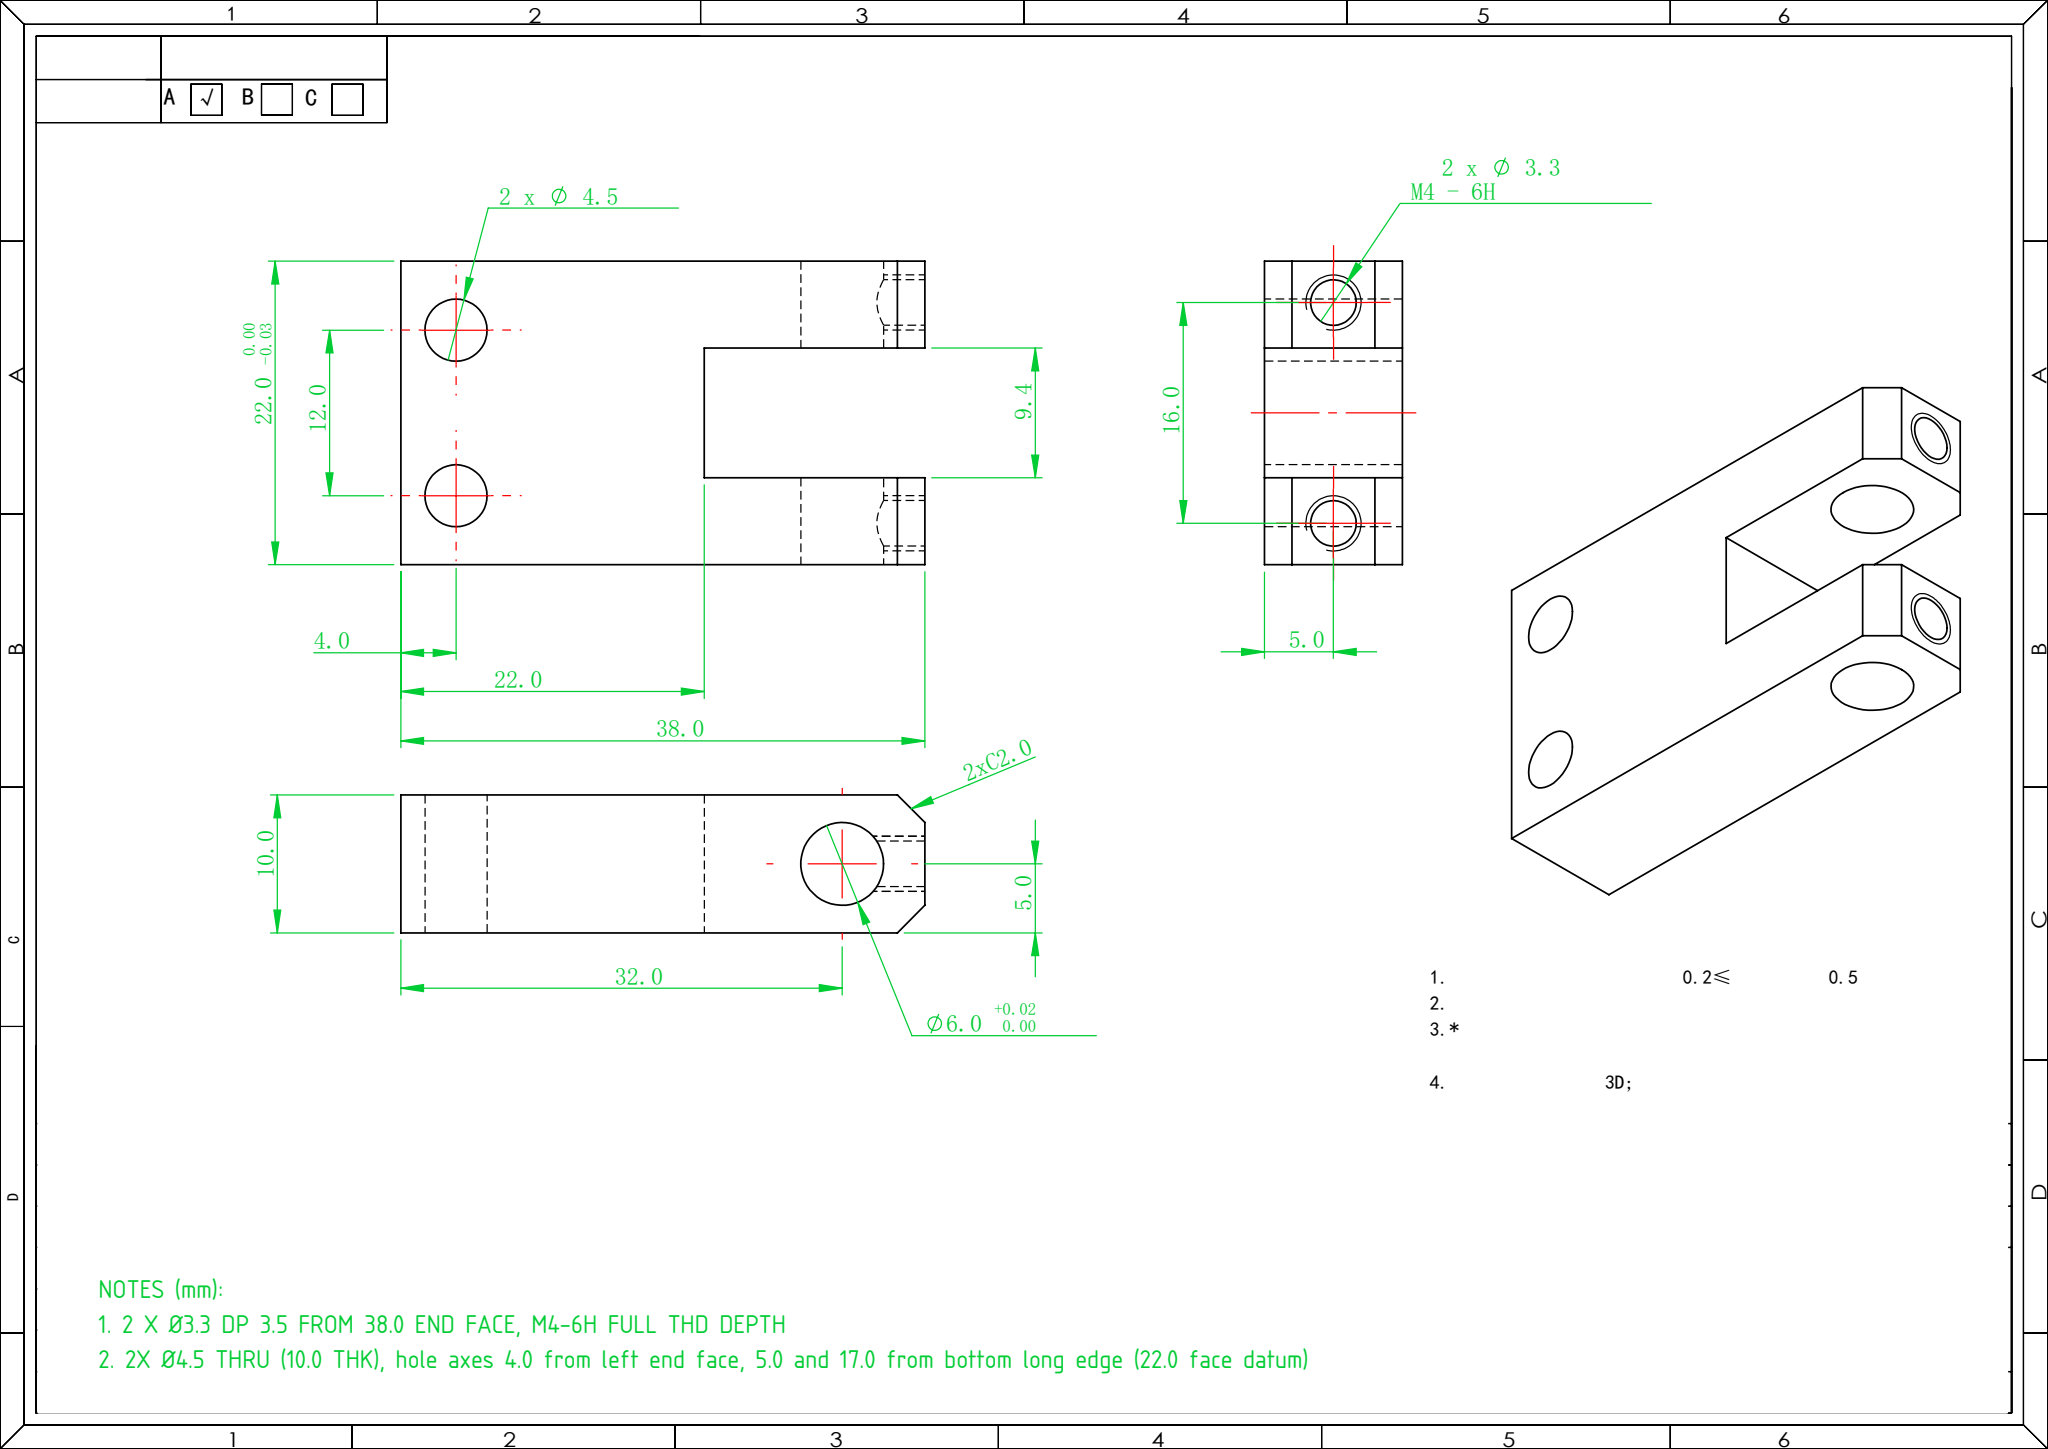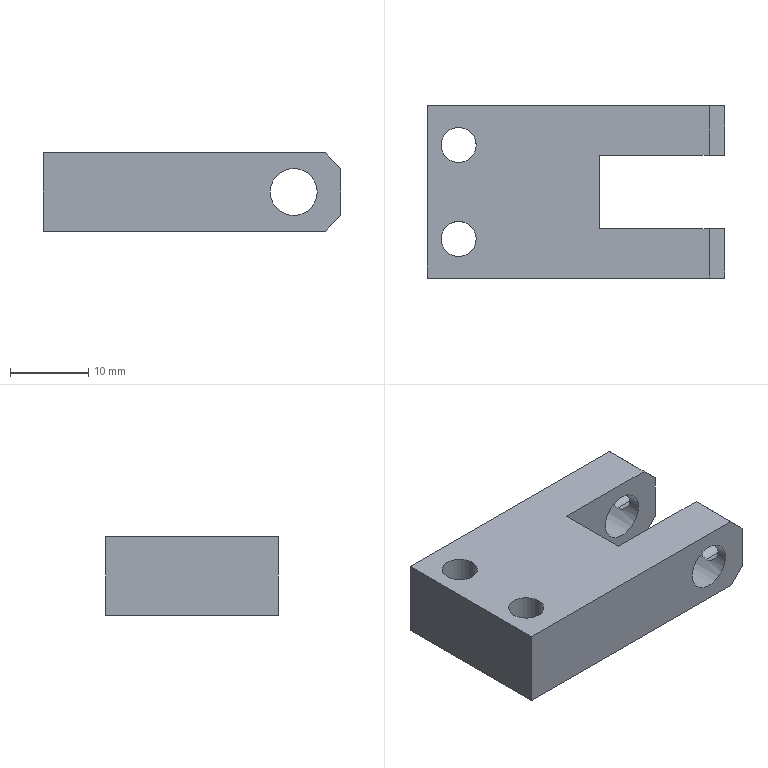Part | SolidWorks | mm | 1 solid | 26 faces | box 38 x 22 x 10 mm | volume 6078 mm3 | plane 14 | cylinder 12 | commonest cylinder face diameters 4.5 x4 3.3 x4 6 x4
Drawing notes:
2 X Ø3.3 DP 3.5 FROM 38.0 END FACE, M4-6H FULL THD DEPTH | from the solid: cylinders [3.3,"x",[null,3.0,5.0],3.49] and [3.3,"x",[null,19.0,5.0],3.49]; blind from x=38.0 face
2X Ø4.5 THRU (10.0 THK), hole axes 4.0 from left end face, 5.0 and 17.0 from bottom long edge (22.0 face datum) | from the solid: cylinders [4.5, axis z, pos (4.0, 5.0) and (4.0, 17.0), length 10.0] with bbox_xyz z = 10.0
STEP:
#1=CARTESIAN_POINT('',(-12.75,-6.,0.));
#2=VERTEX_POINT('',#1);
#3=CARTESIAN_POINT('',(-17.25,-6.,0.));
#4=VERTEX_POINT('',#3);
#5=CARTESIAN_POINT('',(-15.,-6.,0.));
#6=DIRECTION('',(0.,0.,-1.));
#7=DIRECTION('',(-1.,0.,0.));
#8=AXIS2_PLACEMENT_3D('',#5,#6,#7);
#9=CIRCLE('',#8,2.25);
#10=EDGE_CURVE('',#2,#4,#9,.T.);
#11=ORIENTED_EDGE('',*,*,#10,.T.);
#12=CARTESIAN_POINT('',(-17.25,-6.,10.));
#13=VERTEX_POINT('',#12);
#14=CARTESIAN_POINT('',(-17.25,-6.,10.));
#15=DIRECTION('',(0.,0.,1.));
#16=VECTOR('',#15,1000.);
#17=LINE('',#14,#16);
#18=EDGE_CURVE('',#4,#13,#17,.T.);
#19=ORIENTED_EDGE('',*,*,#18,.T.);
#20=CARTESIAN_POINT('',(-12.75,-6.,10.));
#21=VERTEX_POINT('',#20);
#22=CARTESIAN_POINT('',(-15.,-6.,10.));
#23=DIRECTION('',(0.,0.,1.));
#24=DIRECTION('',(1.,0.,0.));
#25=AXIS2_PLACEMENT_3D('',#22,#23,#24);
#26=CIRCLE('',#25,2.25);
#27=EDGE_CURVE('',#13,#21,#26,.T.);
#28=ORIENTED_EDGE('',*,*,#27,.T.);
#29=CARTESIAN_POINT('',(-12.75,-6.,10.));
#30=DIRECTION('',(0.,0.,1.));
#31=VECTOR('',#30,1000.);
#32=LINE('',#29,#31);
#33=EDGE_CURVE('',#2,#21,#32,.T.);
#34=ORIENTED_EDGE('',*,*,#33,.F.);
#35=EDGE_LOOP('',(#11,#19,#28,#34));
#36=FACE_OUTER_BOUND('',#35,.T.);
#37=CARTESIAN_POINT('',(-15.,-6.,10.));
#38=DIRECTION('',(0.,0.,1.));
#39=DIRECTION('',(1.,0.,0.));
#40=AXIS2_PLACEMENT_3D('',#37,#38,#39);
#41=CYLINDRICAL_SURFACE('',#40,2.25);
#42=ADVANCED_FACE('',(#36),#41,.F.);
#43=CARTESIAN_POINT('',(-12.75,6.,0.));
#44=VERTEX_POINT('',#43);
#45=CARTESIAN_POINT('',(-17.25,6.,0.));
#46=VERTEX_POINT('',#45);
#47=CARTESIAN_POINT('',(-15.,6.,0.));
#48=DIRECTION('',(0.,0.,-1.));
#49=DIRECTION('',(-1.,0.,0.));
#50=AXIS2_PLACEMENT_3D('',#47,#48,#49);
#51=CIRCLE('',#50,2.25);
#52=EDGE_CURVE('',#44,#46,#51,.T.);
#53=ORIENTED_EDGE('',*,*,#52,.T.);
#54=CARTESIAN_POINT('',(-17.25,6.,10.));
#55=VERTEX_POINT('',#54);
#56=CARTESIAN_POINT('',(-17.25,6.,10.));
#57=DIRECTION('',(0.,0.,1.));
#58=VECTOR('',#57,1000.);
#59=LINE('',#56,#58);
#60=EDGE_CURVE('',#46,#55,#59,.T.);
#61=ORIENTED_EDGE('',*,*,#60,.T.);
#62=CARTESIAN_POINT('',(-12.75,6.,10.));
#63=VERTEX_POINT('',#62);
#64=CARTESIAN_POINT('',(-15.,6.,10.));
#65=DIRECTION('',(0.,0.,1.));
#66=DIRECTION('',(1.,0.,0.));
#67=AXIS2_PLACEMENT_3D('',#64,#65,#66);
#68=CIRCLE('',#67,2.25);
#69=EDGE_CURVE('',#55,#63,#68,.T.);
#70=ORIENTED_EDGE('',*,*,#69,.T.);
#71=CARTESIAN_POINT('',(-12.75,6.,10.));
#72=DIRECTION('',(0.,0.,1.));
#73=VECTOR('',#72,1000.);
#74=LINE('',#71,#73);
#75=EDGE_CURVE('',#44,#63,#74,.T.);
#76=ORIENTED_EDGE('',*,*,#75,.F.);
#77=EDGE_LOOP('',(#53,#61,#70,#76));
#78=FACE_OUTER_BOUND('',#77,.T.);
#79=CARTESIAN_POINT('',(-15.,6.,10.));
#80=DIRECTION('',(0.,0.,1.));
#81=DIRECTION('',(1.,0.,0.));
#82=AXIS2_PLACEMENT_3D('',#79,#80,#81);
#83=CYLINDRICAL_SURFACE('',#82,2.25);
#84=ADVANCED_FACE('',(#78),#83,.F.);
#85=CARTESIAN_POINT('',(15.505,-8.,6.65));
#86=VERTEX_POINT('',#85);
#87=CARTESIAN_POINT('',(16.,-9.65,5.));
#88=VERTEX_POINT('',#87);
#89=CARTESIAN_POINT('',(15.505,-8.,6.65));
#90=CARTESIAN_POINT('',(15.505,-8.11,6.65));
#91=CARTESIAN_POINT('',(15.513,-8.222,6.639));
#92=CARTESIAN_POINT('',(15.541,-8.436,6.595));
#93=CARTESIAN_POINT('',(15.561,-8.541,6.563));
#94=CARTESIAN_POINT('',(15.635,-8.839,6.437));
#95=CARTESIAN_POINT('',(15.701,-9.018,6.316));
#96=CARTESIAN_POINT('',(15.827,-9.316,6.018));
#97=CARTESIAN_POINT('',(15.888,-9.438,5.837));
#98=CARTESIAN_POINT('',(15.953,-9.563,5.54));
#99=CARTESIAN_POINT('',(15.97,-9.596,5.434));
#100=CARTESIAN_POINT('',(15.994,-9.639,5.219));
#101=CARTESIAN_POINT('',(16.,-9.65,5.11));
#102=CARTESIAN_POINT('',(16.,-9.65,5.));
#103=B_SPLINE_CURVE_WITH_KNOTS('',3,(#89,#90,#91,#92,#93,#94,#95,#96,#97,#98,#99,#100,#101,#102),.UNSPECIFIED.,.F.,.F.,(4,2,2,2,2,2,4),(0.002637,0.002966,0.003296,0.003954,0.004612,0.004941,0.00527),.UNSPECIFIED.);
#104=EDGE_CURVE('',#86,#88,#103,.T.);
#105=ORIENTED_EDGE('',*,*,#104,.F.);
#106=CARTESIAN_POINT('',(19.,-8.,6.65));
#107=VERTEX_POINT('',#106);
#108=CARTESIAN_POINT('',(19.,-8.,6.65));
#109=DIRECTION('',(1.,0.,0.));
#110=VECTOR('',#109,1000.);
#111=LINE('',#108,#110);
#112=EDGE_CURVE('',#86,#107,#111,.T.);
#113=ORIENTED_EDGE('',*,*,#112,.T.);
#114=CARTESIAN_POINT('',(19.,-8.,3.35));
#115=VERTEX_POINT('',#114);
#116=CARTESIAN_POINT('',(19.,-8.,5.));
#117=DIRECTION('',(1.,0.,0.));
#118=DIRECTION('',(0.,0.,-1.));
#119=AXIS2_PLACEMENT_3D('',#116,#117,#118);
#120=CIRCLE('',#119,1.65);
#121=EDGE_CURVE('',#107,#115,#120,.T.);
#122=ORIENTED_EDGE('',*,*,#121,.T.);
#123=CARTESIAN_POINT('',(15.505,-8.,3.35));
#124=VERTEX_POINT('',#123);
#125=CARTESIAN_POINT('',(19.,-8.,3.35));
#126=DIRECTION('',(1.,0.,0.));
#127=VECTOR('',#126,1000.);
#128=LINE('',#125,#127);
#129=EDGE_CURVE('',#124,#115,#128,.T.);
#130=ORIENTED_EDGE('',*,*,#129,.F.);
#131=CARTESIAN_POINT('',(16.,-9.65,5.));
#132=CARTESIAN_POINT('',(16.,-9.65,4.89));
#133=CARTESIAN_POINT('',(15.994,-9.639,4.778));
#134=CARTESIAN_POINT('',(15.97,-9.595,4.564));
#135=CARTESIAN_POINT('',(15.953,-9.563,4.459));
#136=CARTESIAN_POINT('',(15.909,-9.478,4.258));
#137=CARTESIAN_POINT('',(15.883,-9.427,4.164));
#138=CARTESIAN_POINT('',(15.826,-9.307,3.988));
#139=CARTESIAN_POINT('',(15.794,-9.239,3.905));
#140=CARTESIAN_POINT('',(15.7,-9.014,3.682));
#141=CARTESIAN_POINT('',(15.634,-8.834,3.561));
#142=CARTESIAN_POINT('',(15.537,-8.44,3.396));
#143=CARTESIAN_POINT('',(15.505,-8.219,3.35));
#144=CARTESIAN_POINT('',(15.505,-8.,3.35));
#145=B_SPLINE_CURVE_WITH_KNOTS('',3,(#131,#132,#133,#134,#135,#136,#137,#138,#139,#140,#141,#142,#143,#144),.UNSPECIFIED.,.F.,.F.,(4,2,2,2,2,2,4),(0.00527,0.005599,0.005928,0.006257,0.006586,0.007244,0.007902),.UNSPECIFIED.);
#146=EDGE_CURVE('',#88,#124,#145,.T.);
#147=ORIENTED_EDGE('',*,*,#146,.F.);
#148=EDGE_LOOP('',(#105,#113,#122,#130,#147));
#149=FACE_OUTER_BOUND('',#148,.T.);
#150=CARTESIAN_POINT('',(19.,-8.,5.));
#151=DIRECTION('',(1.,0.,0.));
#152=DIRECTION('',(0.,0.,-1.));
#153=AXIS2_PLACEMENT_3D('',#150,#151,#152);
#154=CYLINDRICAL_SURFACE('',#153,1.65);
#155=ADVANCED_FACE('',(#149),#154,.F.);
#156=CARTESIAN_POINT('',(15.505,8.,6.65));
#157=VERTEX_POINT('',#156);
#158=CARTESIAN_POINT('',(16.,6.35,5.));
#159=VERTEX_POINT('',#158);
#160=CARTESIAN_POINT('',(15.505,8.,6.65));
#161=CARTESIAN_POINT('',(15.505,7.89,6.65));
#162=CARTESIAN_POINT('',(15.513,7.778,6.639));
#163=CARTESIAN_POINT('',(15.541,7.564,6.595));
#164=CARTESIAN_POINT('',(15.561,7.459,6.563));
#165=CARTESIAN_POINT('',(15.635,7.161,6.437));
#166=CARTESIAN_POINT('',(15.701,6.982,6.316));
#167=CARTESIAN_POINT('',(15.827,6.684,6.018));
#168=CARTESIAN_POINT('',(15.888,6.562,5.837));
#169=CARTESIAN_POINT('',(15.953,6.437,5.54));
#170=CARTESIAN_POINT('',(15.97,6.404,5.434));
#171=CARTESIAN_POINT('',(15.994,6.361,5.219));
#172=CARTESIAN_POINT('',(16.,6.35,5.11));
#173=CARTESIAN_POINT('',(16.,6.35,5.));
#174=B_SPLINE_CURVE_WITH_KNOTS('',3,(#160,#161,#162,#163,#164,#165,#166,#167,#168,#169,#170,#171,#172,#173),.UNSPECIFIED.,.F.,.F.,(4,2,2,2,2,2,4),(0.002637,0.002966,0.003296,0.003954,0.004612,0.004941,0.00527),.UNSPECIFIED.);
#175=EDGE_CURVE('',#157,#159,#174,.T.);
#176=ORIENTED_EDGE('',*,*,#175,.F.);
#177=CARTESIAN_POINT('',(19.,8.,6.65));
#178=VERTEX_POINT('',#177);
#179=CARTESIAN_POINT('',(19.,8.,6.65));
#180=DIRECTION('',(1.,0.,0.));
#181=VECTOR('',#180,1000.);
#182=LINE('',#179,#181);
#183=EDGE_CURVE('',#157,#178,#182,.T.);
#184=ORIENTED_EDGE('',*,*,#183,.T.);
#185=CARTESIAN_POINT('',(19.,8.,3.35));
#186=VERTEX_POINT('',#185);
#187=CARTESIAN_POINT('',(19.,8.,5.));
#188=DIRECTION('',(1.,0.,0.));
#189=DIRECTION('',(0.,0.,-1.));
#190=AXIS2_PLACEMENT_3D('',#187,#188,#189);
#191=CIRCLE('',#190,1.65);
#192=EDGE_CURVE('',#178,#186,#191,.T.);
#193=ORIENTED_EDGE('',*,*,#192,.T.);
#194=CARTESIAN_POINT('',(15.505,8.,3.35));
#195=VERTEX_POINT('',#194);
#196=CARTESIAN_POINT('',(19.,8.,3.35));
#197=DIRECTION('',(1.,0.,0.));
#198=VECTOR('',#197,1000.);
#199=LINE('',#196,#198);
#200=EDGE_CURVE('',#195,#186,#199,.T.);
#201=ORIENTED_EDGE('',*,*,#200,.F.);
#202=CARTESIAN_POINT('',(16.,6.35,5.));
#203=CARTESIAN_POINT('',(16.,6.35,4.89));
#204=CARTESIAN_POINT('',(15.994,6.361,4.778));
#205=CARTESIAN_POINT('',(15.97,6.405,4.564));
#206=CARTESIAN_POINT('',(15.953,6.437,4.459));
#207=CARTESIAN_POINT('',(15.909,6.522,4.258));
#208=CARTESIAN_POINT('',(15.883,6.573,4.164));
#209=CARTESIAN_POINT('',(15.826,6.693,3.988));
#210=CARTESIAN_POINT('',(15.794,6.761,3.905));
#211=CARTESIAN_POINT('',(15.7,6.986,3.682));
#212=CARTESIAN_POINT('',(15.634,7.166,3.561));
#213=CARTESIAN_POINT('',(15.537,7.56,3.396));
#214=CARTESIAN_POINT('',(15.505,7.781,3.35));
#215=CARTESIAN_POINT('',(15.505,8.,3.35));
#216=B_SPLINE_CURVE_WITH_KNOTS('',3,(#202,#203,#204,#205,#206,#207,#208,#209,#210,#211,#212,#213,#214,#215),.UNSPECIFIED.,.F.,.F.,(4,2,2,2,2,2,4),(0.00527,0.005599,0.005928,0.006257,0.006586,0.007244,0.007902),.UNSPECIFIED.);
#217=EDGE_CURVE('',#159,#195,#216,.T.);
#218=ORIENTED_EDGE('',*,*,#217,.F.);
#219=EDGE_LOOP('',(#176,#184,#193,#201,#218));
#220=FACE_OUTER_BOUND('',#219,.T.);
#221=CARTESIAN_POINT('',(19.,8.,5.));
#222=DIRECTION('',(1.,0.,0.));
#223=DIRECTION('',(0.,0.,-1.));
#224=AXIS2_PLACEMENT_3D('',#221,#222,#223);
#225=CYLINDRICAL_SURFACE('',#224,1.65);
#226=ADVANCED_FACE('',(#220),#225,.F.);
#227=CARTESIAN_POINT('',(10.,-4.7,5.));
#228=VERTEX_POINT('',#227);
#229=CARTESIAN_POINT('',(16.,-4.7,5.));
#230=VERTEX_POINT('',#229);
#231=CARTESIAN_POINT('',(13.,-4.7,5.));
#232=DIRECTION('',(0.,-1.,0.));
#233=DIRECTION('',(0.,0.,-1.));
#234=AXIS2_PLACEMENT_3D('',#231,#232,#233);
#235=CIRCLE('',#234,3.);
#236=EDGE_CURVE('',#228,#230,#235,.T.);
#237=ORIENTED_EDGE('',*,*,#236,.F.);
#238=CARTESIAN_POINT('',(10.,-11.,5.));
#239=VERTEX_POINT('',#238);
#240=CARTESIAN_POINT('',(10.,11.,5.));
#241=DIRECTION('',(0.,-1.,0.));
#242=VECTOR('',#241,1000.);
#243=LINE('',#240,#242);
#244=EDGE_CURVE('',#228,#239,#243,.T.);
#245=ORIENTED_EDGE('',*,*,#244,.T.);
#246=CARTESIAN_POINT('',(16.,-11.,5.));
#247=VERTEX_POINT('',#246);
#248=CARTESIAN_POINT('',(13.,-11.,5.));
#249=DIRECTION('',(0.,-1.,0.));
#250=DIRECTION('',(1.,0.,0.));
#251=AXIS2_PLACEMENT_3D('',#248,#249,#250);
#252=CIRCLE('',#251,3.);
#253=EDGE_CURVE('',#239,#247,#252,.T.);
#254=ORIENTED_EDGE('',*,*,#253,.T.);
#255=CARTESIAN_POINT('',(16.,11.,5.));
#256=DIRECTION('',(0.,-1.,0.));
#257=VECTOR('',#256,1000.);
#258=LINE('',#255,#257);
#259=EDGE_CURVE('',#88,#247,#258,.T.);
#260=ORIENTED_EDGE('',*,*,#259,.F.);
#261=ORIENTED_EDGE('',*,*,#146,.T.);
#262=CARTESIAN_POINT('',(16.,-6.35,5.));
#263=VERTEX_POINT('',#262);
#264=CARTESIAN_POINT('',(15.505,-8.,3.35));
#265=CARTESIAN_POINT('',(15.505,-7.89,3.35));
#266=CARTESIAN_POINT('',(15.513,-7.779,3.361));
#267=CARTESIAN_POINT('',(15.541,-7.565,3.405));
#268=CARTESIAN_POINT('',(15.561,-7.461,3.437));
#269=CARTESIAN_POINT('',(15.61,-7.261,3.521));
#270=CARTESIAN_POINT('',(15.639,-7.167,3.572));
#271=CARTESIAN_POINT('',(15.7,-6.992,3.69));
#272=CARTESIAN_POINT('',(15.732,-6.909,3.758));
#273=CARTESIAN_POINT('',(15.795,-6.76,3.907));
#274=CARTESIAN_POINT('',(15.826,-6.692,3.988));
#275=CARTESIAN_POINT('',(15.883,-6.573,4.165));
#276=CARTESIAN_POINT('',(15.909,-6.521,4.26));
#277=CARTESIAN_POINT('',(15.974,-6.396,4.557));
#278=CARTESIAN_POINT('',(16.,-6.35,4.778));
#279=CARTESIAN_POINT('',(16.,-6.35,5.));
#280=B_SPLINE_CURVE_WITH_KNOTS('',3,(#264,#265,#266,#267,#268,#269,#270,#271,#272,#273,#274,#275,#276,#277,#278,#279),.UNSPECIFIED.,.F.,.F.,(4,2,2,2,2,2,2,4),(0.007902,0.00823,0.008558,0.008887,0.009215,0.009543,0.009871,0.01053),.UNSPECIFIED.);
#281=EDGE_CURVE('',#124,#263,#280,.T.);
#282=ORIENTED_EDGE('',*,*,#281,.T.);
#283=CARTESIAN_POINT('',(16.,11.,5.));
#284=DIRECTION('',(0.,-1.,0.));
#285=VECTOR('',#284,1000.);
#286=LINE('',#283,#285);
#287=EDGE_CURVE('',#230,#263,#286,.T.);
#288=ORIENTED_EDGE('',*,*,#287,.F.);
#289=EDGE_LOOP('',(#237,#245,#254,#260,#261,#282,#288));
#290=FACE_OUTER_BOUND('',#289,.T.);
#291=CARTESIAN_POINT('',(13.,11.,5.));
#292=DIRECTION('',(0.,-1.,0.));
#293=DIRECTION('',(1.,0.,0.));
#294=AXIS2_PLACEMENT_3D('',#291,#292,#293);
#295=CYLINDRICAL_SURFACE('',#294,3.);
#296=ADVANCED_FACE('',(#290),#295,.F.);
#297=CARTESIAN_POINT('',(10.,11.,5.));
#298=VERTEX_POINT('',#297);
#299=CARTESIAN_POINT('',(16.,11.,5.));
#300=VERTEX_POINT('',#299);
#301=CARTESIAN_POINT('',(13.,11.,5.));
#302=DIRECTION('',(0.,-1.,0.));
#303=DIRECTION('',(1.,0.,0.));
#304=AXIS2_PLACEMENT_3D('',#301,#302,#303);
#305=CIRCLE('',#304,3.);
#306=EDGE_CURVE('',#298,#300,#305,.T.);
#307=ORIENTED_EDGE('',*,*,#306,.F.);
#308=CARTESIAN_POINT('',(10.,4.7,5.));
#309=VERTEX_POINT('',#308);
#310=CARTESIAN_POINT('',(10.,11.,5.));
#311=DIRECTION('',(0.,-1.,0.));
#312=VECTOR('',#311,1000.);
#313=LINE('',#310,#312);
#314=EDGE_CURVE('',#298,#309,#313,.T.);
#315=ORIENTED_EDGE('',*,*,#314,.T.);
#316=CARTESIAN_POINT('',(16.,4.7,5.));
#317=VERTEX_POINT('',#316);
#318=CARTESIAN_POINT('',(13.,4.7,5.));
#319=DIRECTION('',(0.,1.,0.));
#320=DIRECTION('',(0.,0.,1.));
#321=AXIS2_PLACEMENT_3D('',#318,#319,#320);
#322=CIRCLE('',#321,3.);
#323=EDGE_CURVE('',#317,#309,#322,.T.);
#324=ORIENTED_EDGE('',*,*,#323,.F.);
#325=CARTESIAN_POINT('',(16.,11.,5.));
#326=DIRECTION('',(0.,-1.,0.));
#327=VECTOR('',#326,1000.);
#328=LINE('',#325,#327);
#329=EDGE_CURVE('',#159,#317,#328,.T.);
#330=ORIENTED_EDGE('',*,*,#329,.F.);
#331=ORIENTED_EDGE('',*,*,#217,.T.);
#332=CARTESIAN_POINT('',(16.,9.65,5.));
#333=VERTEX_POINT('',#332);
#334=CARTESIAN_POINT('',(15.505,8.,3.35));
#335=CARTESIAN_POINT('',(15.505,8.11,3.35));
#336=CARTESIAN_POINT('',(15.513,8.221,3.361));
#337=CARTESIAN_POINT('',(15.541,8.435,3.405));
#338=CARTESIAN_POINT('',(15.561,8.539,3.437));
#339=CARTESIAN_POINT('',(15.61,8.739,3.521));
#340=CARTESIAN_POINT('',(15.639,8.833,3.572));
#341=CARTESIAN_POINT('',(15.7,9.008,3.69));
#342=CARTESIAN_POINT('',(15.732,9.091,3.758));
#343=CARTESIAN_POINT('',(15.795,9.24,3.907));
#344=CARTESIAN_POINT('',(15.826,9.308,3.988));
#345=CARTESIAN_POINT('',(15.883,9.427,4.165));
#346=CARTESIAN_POINT('',(15.909,9.479,4.26));
#347=CARTESIAN_POINT('',(15.974,9.604,4.557));
#348=CARTESIAN_POINT('',(16.,9.65,4.778));
#349=CARTESIAN_POINT('',(16.,9.65,5.));
#350=B_SPLINE_CURVE_WITH_KNOTS('',3,(#334,#335,#336,#337,#338,#339,#340,#341,#342,#343,#344,#345,#346,#347,#348,#349),.UNSPECIFIED.,.F.,.F.,(4,2,2,2,2,2,2,4),(0.007902,0.00823,0.008558,0.008887,0.009215,0.009543,0.009871,0.01053),.UNSPECIFIED.);
#351=EDGE_CURVE('',#195,#333,#350,.T.);
#352=ORIENTED_EDGE('',*,*,#351,.T.);
#353=CARTESIAN_POINT('',(16.,11.,5.));
#354=DIRECTION('',(0.,-1.,0.));
#355=VECTOR('',#354,1000.);
#356=LINE('',#353,#355);
#357=EDGE_CURVE('',#300,#333,#356,.T.);
#358=ORIENTED_EDGE('',*,*,#357,.F.);
#359=EDGE_LOOP('',(#307,#315,#324,#330,#331,#352,#358));
#360=FACE_OUTER_BOUND('',#359,.T.);
#361=CARTESIAN_POINT('',(13.,11.,5.));
#362=DIRECTION('',(0.,-1.,0.));
#363=DIRECTION('',(1.,0.,0.));
#364=AXIS2_PLACEMENT_3D('',#361,#362,#363);
#365=CYLINDRICAL_SURFACE('',#364,3.);
#366=ADVANCED_FACE('',(#360),#365,.F.);
#367=CARTESIAN_POINT('',(3.,4.7,10.));
#368=VERTEX_POINT('',#367);
#369=CARTESIAN_POINT('',(17.,4.7,10.));
#370=VERTEX_POINT('',#369);
#371=CARTESIAN_POINT('',(35.,4.7,10.));
#372=DIRECTION('',(1.,0.,0.));
#373=VECTOR('',#372,1000.);
#374=LINE('',#371,#373);
#375=EDGE_CURVE('',#368,#370,#374,.T.);
#376=ORIENTED_EDGE('',*,*,#375,.T.);
#377=CARTESIAN_POINT('',(17.,11.,10.));
#378=VERTEX_POINT('',#377);
#379=CARTESIAN_POINT('',(17.,0.,10.));
#380=DIRECTION('',(0.,1.,0.));
#381=VECTOR('',#380,1000.);
#382=LINE('',#379,#381);
#383=EDGE_CURVE('',#370,#378,#382,.T.);
#384=ORIENTED_EDGE('',*,*,#383,.T.);
#385=CARTESIAN_POINT('',(-19.,11.,10.));
#386=VERTEX_POINT('',#385);
#387=CARTESIAN_POINT('',(19.,11.,10.));
#388=DIRECTION('',(-1.,-0.,0.));
#389=VECTOR('',#388,1000.);
#390=LINE('',#387,#389);
#391=EDGE_CURVE('',#378,#386,#390,.T.);
#392=ORIENTED_EDGE('',*,*,#391,.T.);
#393=CARTESIAN_POINT('',(-19.,-11.,10.));
#394=VERTEX_POINT('',#393);
#395=CARTESIAN_POINT('',(-19.,11.,10.));
#396=DIRECTION('',(0.,-1.,0.));
#397=VECTOR('',#396,1000.);
#398=LINE('',#395,#397);
#399=EDGE_CURVE('',#386,#394,#398,.T.);
#400=ORIENTED_EDGE('',*,*,#399,.T.);
#401=CARTESIAN_POINT('',(17.,-11.,10.));
#402=VERTEX_POINT('',#401);
#403=CARTESIAN_POINT('',(19.,-11.,10.));
#404=DIRECTION('',(1.,0.,0.));
#405=VECTOR('',#404,1000.);
#406=LINE('',#403,#405);
#407=EDGE_CURVE('',#394,#402,#406,.T.);
#408=ORIENTED_EDGE('',*,*,#407,.T.);
#409=CARTESIAN_POINT('',(17.,-4.7,10.));
#410=VERTEX_POINT('',#409);
#411=CARTESIAN_POINT('',(17.,0.,10.));
#412=DIRECTION('',(0.,1.,0.));
#413=VECTOR('',#412,1000.);
#414=LINE('',#411,#413);
#415=EDGE_CURVE('',#402,#410,#414,.T.);
#416=ORIENTED_EDGE('',*,*,#415,.T.);
#417=CARTESIAN_POINT('',(3.,-4.7,10.));
#418=VERTEX_POINT('',#417);
#419=CARTESIAN_POINT('',(35.,-4.7,10.));
#420=DIRECTION('',(-1.,0.,0.));
#421=VECTOR('',#420,1000.);
#422=LINE('',#419,#421);
#423=EDGE_CURVE('',#410,#418,#422,.T.);
#424=ORIENTED_EDGE('',*,*,#423,.T.);
#425=CARTESIAN_POINT('',(3.,4.7,10.));
#426=DIRECTION('',(0.,1.,0.));
#427=VECTOR('',#426,1000.);
#428=LINE('',#425,#427);
#429=EDGE_CURVE('',#418,#368,#428,.T.);
#430=ORIENTED_EDGE('',*,*,#429,.T.);
#431=EDGE_LOOP('',(#376,#384,#392,#400,#408,#416,#424,#430));
#432=FACE_OUTER_BOUND('',#431,.T.);
#433=CARTESIAN_POINT('',(-15.,6.,10.));
#434=DIRECTION('',(0.,0.,1.));
#435=DIRECTION('',(1.,0.,0.));
#436=AXIS2_PLACEMENT_3D('',#433,#434,#435);
#437=CIRCLE('',#436,2.25);
#438=EDGE_CURVE('',#63,#55,#437,.T.);
#439=ORIENTED_EDGE('',*,*,#438,.F.);
#440=ORIENTED_EDGE('',*,*,#69,.F.);
#441=EDGE_LOOP('',(#439,#440));
#442=FACE_BOUND('',#441,.T.);
#443=CARTESIAN_POINT('',(-15.,-6.,10.));
#444=DIRECTION('',(0.,0.,1.));
#445=DIRECTION('',(1.,0.,0.));
#446=AXIS2_PLACEMENT_3D('',#443,#444,#445);
#447=CIRCLE('',#446,2.25);
#448=EDGE_CURVE('',#21,#13,#447,.T.);
#449=ORIENTED_EDGE('',*,*,#448,.F.);
#450=ORIENTED_EDGE('',*,*,#27,.F.);
#451=EDGE_LOOP('',(#449,#450));
#452=FACE_BOUND('',#451,.T.);
#453=CARTESIAN_POINT('',(0.,0.,10.));
#454=DIRECTION('',(0.,0.,-1.));
#455=DIRECTION('',(-1.,0.,0.));
#456=AXIS2_PLACEMENT_3D('',#453,#454,#455);
#457=PLANE('',#456);
#458=ADVANCED_FACE('',(#432,#442,#452),#457,.F.);
#459=CARTESIAN_POINT('',(19.,11.,8.));
#460=VERTEX_POINT('',#459);
#461=CARTESIAN_POINT('',(19.,11.,2.));
#462=VERTEX_POINT('',#461);
#463=CARTESIAN_POINT('',(19.,11.,10.));
#464=DIRECTION('',(0.,0.,-1.));
#465=VECTOR('',#464,1000.);
#466=LINE('',#463,#465);
#467=EDGE_CURVE('',#460,#462,#466,.T.);
#468=ORIENTED_EDGE('',*,*,#467,.F.);
#469=CARTESIAN_POINT('',(19.,4.7,8.));
#470=VERTEX_POINT('',#469);
#471=CARTESIAN_POINT('',(19.,11.,8.));
#472=DIRECTION('',(0.,-1.,0.));
#473=VECTOR('',#472,1000.);
#474=LINE('',#471,#473);
#475=EDGE_CURVE('',#460,#470,#474,.T.);
#476=ORIENTED_EDGE('',*,*,#475,.T.);
#477=CARTESIAN_POINT('',(19.,4.7,2.));
#478=VERTEX_POINT('',#477);
#479=CARTESIAN_POINT('',(19.,4.7,10.));
#480=DIRECTION('',(0.,0.,-1.));
#481=VECTOR('',#480,1000.);
#482=LINE('',#479,#481);
#483=EDGE_CURVE('',#470,#478,#482,.T.);
#484=ORIENTED_EDGE('',*,*,#483,.T.);
#485=CARTESIAN_POINT('',(19.,11.,2.));
#486=DIRECTION('',(0.,1.,0.));
#487=VECTOR('',#486,1000.);
#488=LINE('',#485,#487);
#489=EDGE_CURVE('',#478,#462,#488,.T.);
#490=ORIENTED_EDGE('',*,*,#489,.T.);
#491=EDGE_LOOP('',(#468,#476,#484,#490));
#492=FACE_OUTER_BOUND('',#491,.T.);
#493=CARTESIAN_POINT('',(19.,8.,5.));
#494=DIRECTION('',(1.,0.,0.));
#495=DIRECTION('',(0.,0.,-1.));
#496=AXIS2_PLACEMENT_3D('',#493,#494,#495);
#497=CIRCLE('',#496,1.65);
#498=EDGE_CURVE('',#186,#178,#497,.T.);
#499=ORIENTED_EDGE('',*,*,#498,.F.);
#500=ORIENTED_EDGE('',*,*,#192,.F.);
#501=EDGE_LOOP('',(#499,#500));
#502=FACE_BOUND('',#501,.T.);
#503=CARTESIAN_POINT('',(19.,11.,10.));
#504=DIRECTION('',(-1.,0.,0.));
#505=DIRECTION('',(0.,0.,1.));
#506=AXIS2_PLACEMENT_3D('',#503,#504,#505);
#507=PLANE('',#506);
#508=ADVANCED_FACE('',(#492,#502),#507,.F.);
#509=CARTESIAN_POINT('',(19.,-8.,5.));
#510=DIRECTION('',(1.,0.,0.));
#511=DIRECTION('',(0.,0.,-1.));
#512=AXIS2_PLACEMENT_3D('',#509,#510,#511);
#513=CIRCLE('',#512,1.65);
#514=EDGE_CURVE('',#115,#107,#513,.T.);
#515=ORIENTED_EDGE('',*,*,#514,.F.);
#516=ORIENTED_EDGE('',*,*,#121,.F.);
#517=EDGE_LOOP('',(#515,#516));
#518=FACE_BOUND('',#517,.T.);
#519=CARTESIAN_POINT('',(19.,-11.,8.));
#520=VERTEX_POINT('',#519);
#521=CARTESIAN_POINT('',(19.,-11.,2.));
#522=VERTEX_POINT('',#521);
#523=CARTESIAN_POINT('',(19.,-11.,10.));
#524=DIRECTION('',(0.,0.,-1.));
#525=VECTOR('',#524,1000.);
#526=LINE('',#523,#525);
#527=EDGE_CURVE('',#520,#522,#526,.T.);
#528=ORIENTED_EDGE('',*,*,#527,.T.);
#529=CARTESIAN_POINT('',(19.,-4.7,2.));
#530=VERTEX_POINT('',#529);
#531=CARTESIAN_POINT('',(19.,-4.7,2.));
#532=DIRECTION('',(0.,1.,0.));
#533=VECTOR('',#532,1000.);
#534=LINE('',#531,#533);
#535=EDGE_CURVE('',#522,#530,#534,.T.);
#536=ORIENTED_EDGE('',*,*,#535,.T.);
#537=CARTESIAN_POINT('',(19.,-4.7,8.));
#538=VERTEX_POINT('',#537);
#539=CARTESIAN_POINT('',(19.,-4.7,10.));
#540=DIRECTION('',(0.,0.,1.));
#541=VECTOR('',#540,1000.);
#542=LINE('',#539,#541);
#543=EDGE_CURVE('',#530,#538,#542,.T.);
#544=ORIENTED_EDGE('',*,*,#543,.T.);
#545=CARTESIAN_POINT('',(19.,11.,8.));
#546=DIRECTION('',(0.,-1.,0.));
#547=VECTOR('',#546,1000.);
#548=LINE('',#545,#547);
#549=EDGE_CURVE('',#538,#520,#548,.T.);
#550=ORIENTED_EDGE('',*,*,#549,.T.);
#551=EDGE_LOOP('',(#528,#536,#544,#550));
#552=FACE_OUTER_BOUND('',#551,.T.);
#553=CARTESIAN_POINT('',(19.,11.,10.));
#554=DIRECTION('',(-1.,0.,0.));
#555=DIRECTION('',(0.,0.,1.));
#556=AXIS2_PLACEMENT_3D('',#553,#554,#555);
#557=PLANE('',#556);
#558=ADVANCED_FACE('',(#518,#552),#557,.F.);
#559=CARTESIAN_POINT('',(-19.,11.,0.));
#560=VERTEX_POINT('',#559);
#561=CARTESIAN_POINT('',(-19.,-11.,0.));
#562=VERTEX_POINT('',#561);
#563=CARTESIAN_POINT('',(-19.,11.,0.));
#564=DIRECTION('',(0.,-1.,0.));
#565=VECTOR('',#564,1000.);
#566=LINE('',#563,#565);
#567=EDGE_CURVE('',#560,#562,#566,.T.);
#568=ORIENTED_EDGE('',*,*,#567,.T.);
#569=CARTESIAN_POINT('',(-19.,-11.,10.));
#570=DIRECTION('',(0.,0.,-1.));
#571=VECTOR('',#570,1000.);
#572=LINE('',#569,#571);
#573=EDGE_CURVE('',#394,#562,#572,.T.);
#574=ORIENTED_EDGE('',*,*,#573,.F.);
#575=ORIENTED_EDGE('',*,*,#399,.F.);
#576=CARTESIAN_POINT('',(-19.,11.,10.));
#577=DIRECTION('',(0.,0.,-1.));
#578=VECTOR('',#577,1000.);
#579=LINE('',#576,#578);
#580=EDGE_CURVE('',#386,#560,#579,.T.);
#581=ORIENTED_EDGE('',*,*,#580,.T.);
#582=EDGE_LOOP('',(#568,#574,#575,#581));
#583=FACE_OUTER_BOUND('',#582,.T.);
#584=CARTESIAN_POINT('',(-19.,11.,10.));
#585=DIRECTION('',(1.,0.,0.));
#586=DIRECTION('',(-0.,1.,0.));
#587=AXIS2_PLACEMENT_3D('',#584,#585,#586);
#588=PLANE('',#587);
#589=ADVANCED_FACE('',(#583),#588,.F.);
#590=CARTESIAN_POINT('',(13.,-11.,5.));
#591=DIRECTION('',(0.,-1.,0.));
#592=DIRECTION('',(1.,0.,0.));
#593=AXIS2_PLACEMENT_3D('',#590,#591,#592);
#594=CIRCLE('',#593,3.);
#595=EDGE_CURVE('',#247,#239,#594,.T.);
#596=ORIENTED_EDGE('',*,*,#595,.F.);
#597=ORIENTED_EDGE('',*,*,#253,.F.);
#598=EDGE_LOOP('',(#596,#597));
#599=FACE_BOUND('',#598,.T.);
#600=CARTESIAN_POINT('',(17.,-11.,0.));
#601=VERTEX_POINT('',#600);
#602=CARTESIAN_POINT('',(19.,-11.,0.));
#603=DIRECTION('',(1.,0.,0.));
#604=VECTOR('',#603,1000.);
#605=LINE('',#602,#604);
#606=EDGE_CURVE('',#562,#601,#605,.T.);
#607=ORIENTED_EDGE('',*,*,#606,.T.);
#608=CARTESIAN_POINT('',(19.,-11.,2.));
#609=DIRECTION('',(0.7071,0.,0.7071));
#610=VECTOR('',#609,1000.);
#611=LINE('',#608,#610);
#612=EDGE_CURVE('',#601,#522,#611,.T.);
#613=ORIENTED_EDGE('',*,*,#612,.T.);
#614=ORIENTED_EDGE('',*,*,#527,.F.);
#615=CARTESIAN_POINT('',(17.,-11.,10.));
#616=DIRECTION('',(-0.7071,-0.,0.7071));
#617=VECTOR('',#616,1000.);
#618=LINE('',#615,#617);
#619=EDGE_CURVE('',#520,#402,#618,.T.);
#620=ORIENTED_EDGE('',*,*,#619,.T.);
#621=ORIENTED_EDGE('',*,*,#407,.F.);
#622=ORIENTED_EDGE('',*,*,#573,.T.);
#623=EDGE_LOOP('',(#607,#613,#614,#620,#621,#622));
#624=FACE_OUTER_BOUND('',#623,.T.);
#625=CARTESIAN_POINT('',(19.,-11.,10.));
#626=DIRECTION('',(-0.,1.,0.));
#627=DIRECTION('',(-1.,-0.,0.));
#628=AXIS2_PLACEMENT_3D('',#625,#626,#627);
#629=PLANE('',#628);
#630=ADVANCED_FACE('',(#599,#624),#629,.F.);
#631=CARTESIAN_POINT('',(13.,11.,5.));
#632=DIRECTION('',(0.,-1.,0.));
#633=DIRECTION('',(1.,0.,0.));
#634=AXIS2_PLACEMENT_3D('',#631,#632,#633);
#635=CIRCLE('',#634,3.);
#636=EDGE_CURVE('',#300,#298,#635,.T.);
#637=ORIENTED_EDGE('',*,*,#636,.T.);
#638=ORIENTED_EDGE('',*,*,#306,.T.);
#639=EDGE_LOOP('',(#637,#638));
#640=FACE_BOUND('',#639,.T.);
#641=ORIENTED_EDGE('',*,*,#391,.F.);
#642=CARTESIAN_POINT('',(17.,11.,10.));
#643=DIRECTION('',(0.7071,0.,-0.7071));
#644=VECTOR('',#643,1000.);
#645=LINE('',#642,#644);
#646=EDGE_CURVE('',#378,#460,#645,.T.);
#647=ORIENTED_EDGE('',*,*,#646,.T.);
#648=ORIENTED_EDGE('',*,*,#467,.T.);
#649=CARTESIAN_POINT('',(17.,11.,0.));
#650=VERTEX_POINT('',#649);
#651=CARTESIAN_POINT('',(19.,11.,2.));
#652=DIRECTION('',(-0.7071,-0.,-0.7071));
#653=VECTOR('',#652,1000.);
#654=LINE('',#651,#653);
#655=EDGE_CURVE('',#462,#650,#654,.T.);
#656=ORIENTED_EDGE('',*,*,#655,.T.);
#657=CARTESIAN_POINT('',(19.,11.,0.));
#658=DIRECTION('',(-1.,-0.,0.));
#659=VECTOR('',#658,1000.);
#660=LINE('',#657,#659);
#661=EDGE_CURVE('',#650,#560,#660,.T.);
#662=ORIENTED_EDGE('',*,*,#661,.T.);
#663=ORIENTED_EDGE('',*,*,#580,.F.);
#664=EDGE_LOOP('',(#641,#647,#648,#656,#662,#663));
#665=FACE_OUTER_BOUND('',#664,.T.);
#666=CARTESIAN_POINT('',(19.,11.,10.));
#667=DIRECTION('',(0.,-1.,0.));
#668=DIRECTION('',(1.,0.,0.));
#669=AXIS2_PLACEMENT_3D('',#666,#667,#668);
#670=PLANE('',#669);
#671=ADVANCED_FACE('',(#640,#665),#670,.F.);
#672=ORIENTED_EDGE('',*,*,#10,.F.);
#673=CARTESIAN_POINT('',(-15.,-6.,0.));
#674=DIRECTION('',(0.,0.,-1.));
#675=DIRECTION('',(-1.,0.,0.));
#676=AXIS2_PLACEMENT_3D('',#673,#674,#675);
#677=CIRCLE('',#676,2.25);
#678=EDGE_CURVE('',#4,#2,#677,.T.);
#679=ORIENTED_EDGE('',*,*,#678,.F.);
#680=EDGE_LOOP('',(#672,#679));
#681=FACE_BOUND('',#680,.T.);
#682=ORIENTED_EDGE('',*,*,#52,.F.);
#683=CARTESIAN_POINT('',(-15.,6.,0.));
#684=DIRECTION('',(0.,0.,-1.));
#685=DIRECTION('',(-1.,0.,0.));
#686=AXIS2_PLACEMENT_3D('',#683,#684,#685);
#687=CIRCLE('',#686,2.25);
#688=EDGE_CURVE('',#46,#44,#687,.T.);
#689=ORIENTED_EDGE('',*,*,#688,.F.);
#690=EDGE_LOOP('',(#682,#689));
#691=FACE_BOUND('',#690,.T.);
#692=ORIENTED_EDGE('',*,*,#661,.F.);
#693=CARTESIAN_POINT('',(17.,4.7,0.));
#694=VERTEX_POINT('',#693);
#695=CARTESIAN_POINT('',(17.,4.7,0.));
#696=DIRECTION('',(0.,-1.,0.));
#697=VECTOR('',#696,1000.);
#698=LINE('',#695,#697);
#699=EDGE_CURVE('',#650,#694,#698,.T.);
#700=ORIENTED_EDGE('',*,*,#699,.T.);
#701=CARTESIAN_POINT('',(3.,4.7,0.));
#702=VERTEX_POINT('',#701);
#703=CARTESIAN_POINT('',(35.,4.7,0.));
#704=DIRECTION('',(1.,0.,0.));
#705=VECTOR('',#704,1000.);
#706=LINE('',#703,#705);
#707=EDGE_CURVE('',#702,#694,#706,.T.);
#708=ORIENTED_EDGE('',*,*,#707,.F.);
#709=CARTESIAN_POINT('',(3.,-4.7,0.));
#710=VERTEX_POINT('',#709);
#711=CARTESIAN_POINT('',(3.,4.7,0.));
#712=DIRECTION('',(0.,1.,0.));
#713=VECTOR('',#712,1000.);
#714=LINE('',#711,#713);
#715=EDGE_CURVE('',#710,#702,#714,.T.);
#716=ORIENTED_EDGE('',*,*,#715,.F.);
#717=CARTESIAN_POINT('',(17.,-4.7,0.));
#718=VERTEX_POINT('',#717);
#719=CARTESIAN_POINT('',(0.,-4.7,0.));
#720=DIRECTION('',(-1.,0.,0.));
#721=VECTOR('',#720,1000.);
#722=LINE('',#719,#721);
#723=EDGE_CURVE('',#718,#710,#722,.T.);
#724=ORIENTED_EDGE('',*,*,#723,.F.);
#725=CARTESIAN_POINT('',(17.,-11.,0.));
#726=DIRECTION('',(0.,-1.,0.));
#727=VECTOR('',#726,1000.);
#728=LINE('',#725,#727);
#729=EDGE_CURVE('',#718,#601,#728,.T.);
#730=ORIENTED_EDGE('',*,*,#729,.T.);
#731=ORIENTED_EDGE('',*,*,#606,.F.);
#732=ORIENTED_EDGE('',*,*,#567,.F.);
#733=EDGE_LOOP('',(#692,#700,#708,#716,#724,#730,#731,#732));
#734=FACE_OUTER_BOUND('',#733,.T.);
#735=CARTESIAN_POINT('',(0.,0.,0.));
#736=DIRECTION('',(0.,0.,-1.));
#737=DIRECTION('',(-1.,0.,0.));
#738=AXIS2_PLACEMENT_3D('',#735,#736,#737);
#739=PLANE('',#738);
#740=ADVANCED_FACE('',(#681,#691,#734),#739,.T.);
#741=CARTESIAN_POINT('',(13.,-4.7,5.));
#742=DIRECTION('',(0.,-1.,0.));
#743=DIRECTION('',(0.,0.,-1.));
#744=AXIS2_PLACEMENT_3D('',#741,#742,#743);
#745=CIRCLE('',#744,3.);
#746=EDGE_CURVE('',#230,#228,#745,.T.);
#747=ORIENTED_EDGE('',*,*,#746,.T.);
#748=ORIENTED_EDGE('',*,*,#236,.T.);
#749=EDGE_LOOP('',(#747,#748));
#750=FACE_BOUND('',#749,.T.);
#751=ORIENTED_EDGE('',*,*,#543,.F.);
#752=CARTESIAN_POINT('',(19.,-4.7,2.));
#753=DIRECTION('',(-0.7071,0.,-0.7071));
#754=VECTOR('',#753,1000.);
#755=LINE('',#752,#754);
#756=EDGE_CURVE('',#530,#718,#755,.T.);
#757=ORIENTED_EDGE('',*,*,#756,.T.);
#758=ORIENTED_EDGE('',*,*,#723,.T.);
#759=CARTESIAN_POINT('',(3.,-4.7,10.));
#760=DIRECTION('',(0.,0.,-1.));
#761=VECTOR('',#760,1000.);
#762=LINE('',#759,#761);
#763=EDGE_CURVE('',#418,#710,#762,.T.);
#764=ORIENTED_EDGE('',*,*,#763,.F.);
#765=ORIENTED_EDGE('',*,*,#423,.F.);
#766=CARTESIAN_POINT('',(17.,-4.7,10.));
#767=DIRECTION('',(0.7071,0.,-0.7071));
#768=VECTOR('',#767,1000.);
#769=LINE('',#766,#768);
#770=EDGE_CURVE('',#410,#538,#769,.T.);
#771=ORIENTED_EDGE('',*,*,#770,.T.);
#772=EDGE_LOOP('',(#751,#757,#758,#764,#765,#771));
#773=FACE_OUTER_BOUND('',#772,.T.);
#774=CARTESIAN_POINT('',(35.,-4.7,10.));
#775=DIRECTION('',(0.,-1.,0.));
#776=DIRECTION('',(0.,0.,-1.));
#777=AXIS2_PLACEMENT_3D('',#774,#775,#776);
#778=PLANE('',#777);
#779=ADVANCED_FACE('',(#750,#773),#778,.F.);
#780=ORIENTED_EDGE('',*,*,#323,.T.);
#781=CARTESIAN_POINT('',(13.,4.7,5.));
#782=DIRECTION('',(0.,1.,0.));
#783=DIRECTION('',(0.,0.,1.));
#784=AXIS2_PLACEMENT_3D('',#781,#782,#783);
#785=CIRCLE('',#784,3.);
#786=EDGE_CURVE('',#309,#317,#785,.T.);
#787=ORIENTED_EDGE('',*,*,#786,.T.);
#788=EDGE_LOOP('',(#780,#787));
#789=FACE_BOUND('',#788,.T.);
#790=ORIENTED_EDGE('',*,*,#483,.F.);
#791=CARTESIAN_POINT('',(17.,4.7,10.));
#792=DIRECTION('',(-0.7071,0.,0.7071));
#793=VECTOR('',#792,1000.);
#794=LINE('',#791,#793);
#795=EDGE_CURVE('',#470,#370,#794,.T.);
#796=ORIENTED_EDGE('',*,*,#795,.T.);
#797=ORIENTED_EDGE('',*,*,#375,.F.);
#798=CARTESIAN_POINT('',(3.,4.7,10.));
#799=DIRECTION('',(0.,0.,-1.));
#800=VECTOR('',#799,1000.);
#801=LINE('',#798,#800);
#802=EDGE_CURVE('',#368,#702,#801,.T.);
#803=ORIENTED_EDGE('',*,*,#802,.T.);
#804=ORIENTED_EDGE('',*,*,#707,.T.);
#805=CARTESIAN_POINT('',(19.,4.7,2.));
#806=DIRECTION('',(0.7071,0.,0.7071));
#807=VECTOR('',#806,1000.);
#808=LINE('',#805,#807);
#809=EDGE_CURVE('',#694,#478,#808,.T.);
#810=ORIENTED_EDGE('',*,*,#809,.T.);
#811=EDGE_LOOP('',(#790,#796,#797,#803,#804,#810));
#812=FACE_OUTER_BOUND('',#811,.T.);
#813=CARTESIAN_POINT('',(35.,4.7,10.));
#814=DIRECTION('',(0.,1.,0.));
#815=DIRECTION('',(0.,0.,1.));
#816=AXIS2_PLACEMENT_3D('',#813,#814,#815);
#817=PLANE('',#816);
#818=ADVANCED_FACE('',(#789,#812),#817,.F.);
#819=ORIENTED_EDGE('',*,*,#715,.T.);
#820=ORIENTED_EDGE('',*,*,#802,.F.);
#821=ORIENTED_EDGE('',*,*,#429,.F.);
#822=ORIENTED_EDGE('',*,*,#763,.T.);
#823=EDGE_LOOP('',(#819,#820,#821,#822));
#824=FACE_OUTER_BOUND('',#823,.T.);
#825=CARTESIAN_POINT('',(3.,4.7,10.));
#826=DIRECTION('',(-1.,0.,0.));
#827=DIRECTION('',(-0.,-1.,0.));
#828=AXIS2_PLACEMENT_3D('',#825,#826,#827);
#829=PLANE('',#828);
#830=ADVANCED_FACE('',(#824),#829,.F.);
#831=ORIENTED_EDGE('',*,*,#314,.F.);
#832=ORIENTED_EDGE('',*,*,#636,.F.);
#833=ORIENTED_EDGE('',*,*,#357,.T.);
#834=CARTESIAN_POINT('',(16.,9.65,5.));
#835=CARTESIAN_POINT('',(16.,9.65,5.112));
#836=CARTESIAN_POINT('',(15.994,9.639,5.221));
#837=CARTESIAN_POINT('',(15.97,9.595,5.435));
#838=CARTESIAN_POINT('',(15.952,9.562,5.541));
#839=CARTESIAN_POINT('',(15.887,9.436,5.84));
#840=CARTESIAN_POINT('',(15.826,9.314,6.02));
#841=CARTESIAN_POINT('',(15.7,9.015,6.318));
#842=CARTESIAN_POINT('',(15.634,8.836,6.439));
#843=CARTESIAN_POINT('',(15.561,8.539,6.563));
#844=CARTESIAN_POINT('',(15.54,8.433,6.596));
#845=CARTESIAN_POINT('',(15.513,8.219,6.639));
#846=CARTESIAN_POINT('',(15.505,8.11,6.65));
#847=CARTESIAN_POINT('',(15.505,8.,6.65));
#848=B_SPLINE_CURVE_WITH_KNOTS('',3,(#834,#835,#836,#837,#838,#839,#840,#841,#842,#843,#844,#845,#846,#847),.UNSPECIFIED.,.F.,.F.,(4,2,2,2,2,2,4),(0.,0.0003297,0.0006593,0.001319,0.001978,0.002308,0.002637),.UNSPECIFIED.);
#849=EDGE_CURVE('',#333,#157,#848,.T.);
#850=ORIENTED_EDGE('',*,*,#849,.T.);
#851=ORIENTED_EDGE('',*,*,#175,.T.);
#852=ORIENTED_EDGE('',*,*,#329,.T.);
#853=ORIENTED_EDGE('',*,*,#786,.F.);
#854=EDGE_LOOP('',(#831,#832,#833,#850,#851,#852,#853));
#855=FACE_OUTER_BOUND('',#854,.T.);
#856=CARTESIAN_POINT('',(13.,11.,5.));
#857=DIRECTION('',(0.,-1.,0.));
#858=DIRECTION('',(1.,0.,0.));
#859=AXIS2_PLACEMENT_3D('',#856,#857,#858);
#860=CYLINDRICAL_SURFACE('',#859,3.);
#861=ADVANCED_FACE('',(#855),#860,.F.);
#862=ORIENTED_EDGE('',*,*,#244,.F.);
#863=ORIENTED_EDGE('',*,*,#746,.F.);
#864=ORIENTED_EDGE('',*,*,#287,.T.);
#865=CARTESIAN_POINT('',(16.,-6.35,5.));
#866=CARTESIAN_POINT('',(16.,-6.35,5.112));
#867=CARTESIAN_POINT('',(15.994,-6.361,5.221));
#868=CARTESIAN_POINT('',(15.97,-6.405,5.435));
#869=CARTESIAN_POINT('',(15.952,-6.438,5.541));
#870=CARTESIAN_POINT('',(15.887,-6.564,5.84));
#871=CARTESIAN_POINT('',(15.826,-6.686,6.02));
#872=CARTESIAN_POINT('',(15.7,-6.985,6.318));
#873=CARTESIAN_POINT('',(15.634,-7.164,6.439));
#874=CARTESIAN_POINT('',(15.561,-7.461,6.563));
#875=CARTESIAN_POINT('',(15.54,-7.567,6.596));
#876=CARTESIAN_POINT('',(15.513,-7.781,6.639));
#877=CARTESIAN_POINT('',(15.505,-7.89,6.65));
#878=CARTESIAN_POINT('',(15.505,-8.,6.65));
#879=B_SPLINE_CURVE_WITH_KNOTS('',3,(#865,#866,#867,#868,#869,#870,#871,#872,#873,#874,#875,#876,#877,#878),.UNSPECIFIED.,.F.,.F.,(4,2,2,2,2,2,4),(0.,0.0003297,0.0006593,0.001319,0.001978,0.002308,0.002637),.UNSPECIFIED.);
#880=EDGE_CURVE('',#263,#86,#879,.T.);
#881=ORIENTED_EDGE('',*,*,#880,.T.);
#882=ORIENTED_EDGE('',*,*,#104,.T.);
#883=ORIENTED_EDGE('',*,*,#259,.T.);
#884=ORIENTED_EDGE('',*,*,#595,.T.);
#885=EDGE_LOOP('',(#862,#863,#864,#881,#882,#883,#884));
#886=FACE_OUTER_BOUND('',#885,.T.);
#887=CARTESIAN_POINT('',(13.,11.,5.));
#888=DIRECTION('',(0.,-1.,0.));
#889=DIRECTION('',(1.,0.,0.));
#890=AXIS2_PLACEMENT_3D('',#887,#888,#889);
#891=CYLINDRICAL_SURFACE('',#890,3.);
#892=ADVANCED_FACE('',(#886),#891,.F.);
#893=ORIENTED_EDGE('',*,*,#795,.F.);
#894=ORIENTED_EDGE('',*,*,#475,.F.);
#895=ORIENTED_EDGE('',*,*,#646,.F.);
#896=ORIENTED_EDGE('',*,*,#383,.F.);
#897=EDGE_LOOP('',(#893,#894,#895,#896));
#898=FACE_OUTER_BOUND('',#897,.T.);
#899=CARTESIAN_POINT('',(17.,0.,10.));
#900=DIRECTION('',(-0.7071,0.,-0.7071));
#901=DIRECTION('',(0.,1.,0.));
#902=AXIS2_PLACEMENT_3D('',#899,#900,#901);
#903=PLANE('',#902);
#904=ADVANCED_FACE('',(#898),#903,.F.);
#905=ORIENTED_EDGE('',*,*,#809,.F.);
#906=ORIENTED_EDGE('',*,*,#699,.F.);
#907=ORIENTED_EDGE('',*,*,#655,.F.);
#908=ORIENTED_EDGE('',*,*,#489,.F.);
#909=EDGE_LOOP('',(#905,#906,#907,#908));
#910=FACE_OUTER_BOUND('',#909,.T.);
#911=CARTESIAN_POINT('',(19.,11.,2.));
#912=DIRECTION('',(0.7071,0.,-0.7071));
#913=DIRECTION('',(0.,-1.,0.));
#914=AXIS2_PLACEMENT_3D('',#911,#912,#913);
#915=PLANE('',#914);
#916=ADVANCED_FACE('',(#910),#915,.T.);
#917=ORIENTED_EDGE('',*,*,#612,.F.);
#918=ORIENTED_EDGE('',*,*,#729,.F.);
#919=ORIENTED_EDGE('',*,*,#756,.F.);
#920=ORIENTED_EDGE('',*,*,#535,.F.);
#921=EDGE_LOOP('',(#917,#918,#919,#920));
#922=FACE_OUTER_BOUND('',#921,.T.);
#923=CARTESIAN_POINT('',(19.,11.,2.));
#924=DIRECTION('',(0.7071,0.,-0.7071));
#925=DIRECTION('',(0.,-1.,0.));
#926=AXIS2_PLACEMENT_3D('',#923,#924,#925);
#927=PLANE('',#926);
#928=ADVANCED_FACE('',(#922),#927,.T.);
#929=ORIENTED_EDGE('',*,*,#619,.F.);
#930=ORIENTED_EDGE('',*,*,#549,.F.);
#931=ORIENTED_EDGE('',*,*,#770,.F.);
#932=ORIENTED_EDGE('',*,*,#415,.F.);
#933=EDGE_LOOP('',(#929,#930,#931,#932));
#934=FACE_OUTER_BOUND('',#933,.T.);
#935=CARTESIAN_POINT('',(17.,0.,10.));
#936=DIRECTION('',(-0.7071,0.,-0.7071));
#937=DIRECTION('',(0.,1.,0.));
#938=AXIS2_PLACEMENT_3D('',#935,#936,#937);
#939=PLANE('',#938);
#940=ADVANCED_FACE('',(#934),#939,.F.);
#941=ORIENTED_EDGE('',*,*,#183,.F.);
#942=ORIENTED_EDGE('',*,*,#849,.F.);
#943=ORIENTED_EDGE('',*,*,#351,.F.);
#944=ORIENTED_EDGE('',*,*,#200,.T.);
#945=ORIENTED_EDGE('',*,*,#498,.T.);
#946=EDGE_LOOP('',(#941,#942,#943,#944,#945));
#947=FACE_OUTER_BOUND('',#946,.T.);
#948=CARTESIAN_POINT('',(19.,8.,5.));
#949=DIRECTION('',(1.,0.,0.));
#950=DIRECTION('',(0.,0.,-1.));
#951=AXIS2_PLACEMENT_3D('',#948,#949,#950);
#952=CYLINDRICAL_SURFACE('',#951,1.65);
#953=ADVANCED_FACE('',(#947),#952,.F.);
#954=ORIENTED_EDGE('',*,*,#112,.F.);
#955=ORIENTED_EDGE('',*,*,#880,.F.);
#956=ORIENTED_EDGE('',*,*,#281,.F.);
#957=ORIENTED_EDGE('',*,*,#129,.T.);
#958=ORIENTED_EDGE('',*,*,#514,.T.);
#959=EDGE_LOOP('',(#954,#955,#956,#957,#958));
#960=FACE_OUTER_BOUND('',#959,.T.);
#961=CARTESIAN_POINT('',(19.,-8.,5.));
#962=DIRECTION('',(1.,0.,0.));
#963=DIRECTION('',(0.,0.,-1.));
#964=AXIS2_PLACEMENT_3D('',#961,#962,#963);
#965=CYLINDRICAL_SURFACE('',#964,1.65);
#966=ADVANCED_FACE('',(#960),#965,.F.);
#967=ORIENTED_EDGE('',*,*,#60,.F.);
#968=ORIENTED_EDGE('',*,*,#688,.T.);
#969=ORIENTED_EDGE('',*,*,#75,.T.);
#970=ORIENTED_EDGE('',*,*,#438,.T.);
#971=EDGE_LOOP('',(#967,#968,#969,#970));
#972=FACE_OUTER_BOUND('',#971,.T.);
#973=CARTESIAN_POINT('',(-15.,6.,10.));
#974=DIRECTION('',(0.,0.,1.));
#975=DIRECTION('',(1.,0.,0.));
#976=AXIS2_PLACEMENT_3D('',#973,#974,#975);
#977=CYLINDRICAL_SURFACE('',#976,2.25);
#978=ADVANCED_FACE('',(#972),#977,.F.);
#979=ORIENTED_EDGE('',*,*,#18,.F.);
#980=ORIENTED_EDGE('',*,*,#678,.T.);
#981=ORIENTED_EDGE('',*,*,#33,.T.);
#982=ORIENTED_EDGE('',*,*,#448,.T.);
#983=EDGE_LOOP('',(#979,#980,#981,#982));
#984=FACE_OUTER_BOUND('',#983,.T.);
#985=CARTESIAN_POINT('',(-15.,-6.,10.));
#986=DIRECTION('',(0.,0.,1.));
#987=DIRECTION('',(1.,0.,0.));
#988=AXIS2_PLACEMENT_3D('',#985,#986,#987);
#989=CYLINDRICAL_SURFACE('',#988,2.25);
#990=ADVANCED_FACE('',(#984),#989,.F.);
#991=CLOSED_SHELL('',(#42,#84,#155,#226,#296,#366,#458,#508,#558,#589,#630,#671,#740,#779,#818,#830,#861,#892,#904,#916,#928,#940,#953,#966,#978,#990));
#992=MANIFOLD_SOLID_BREP('',#991);
#993=CARTESIAN_POINT('',(0.,0.,0.));
#994=DIRECTION('',(0.,0.,1.));
#995=DIRECTION('',(1.,0.,0.));
#996=AXIS2_PLACEMENT_3D('',#993,#994,#995);
#997=(LENGTH_UNIT()NAMED_UNIT(*)SI_UNIT(.MILLI.,.METRE.));
#998=UNCERTAINTY_MEASURE_WITH_UNIT(LENGTH_MEASURE(0.00001),#997,'','');
#999=(NAMED_UNIT(*)PLANE_ANGLE_UNIT()SI_UNIT($,.RADIAN.));
#1000=(NAMED_UNIT(*)SI_UNIT($,.STERADIAN.)SOLID_ANGLE_UNIT());
#1001=(GEOMETRIC_REPRESENTATION_CONTEXT(3)GLOBAL_UNCERTAINTY_ASSIGNED_CONTEXT((#998))GLOBAL_UNIT_ASSIGNED_CONTEXT((#997,#999,#1000))REPRESENTATION_CONTEXT('',''));
#1002=ADVANCED_BREP_SHAPE_REPRESENTATION('',(#992,#996),#1001);